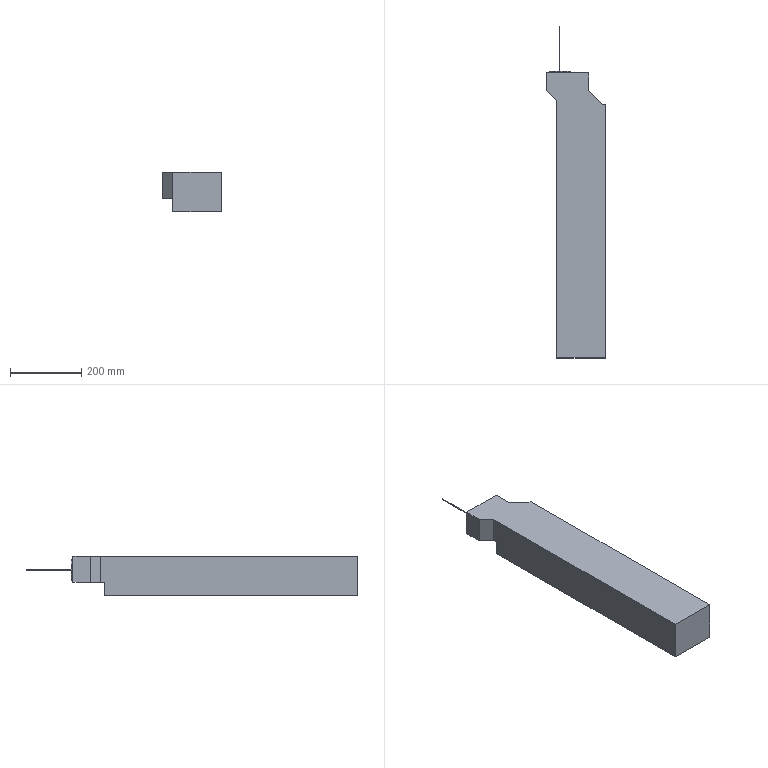Component | SolidWorks | 3120-HSC60-125-1 | 1 solid | 66 faces | volume 11654015 mm3 | cylinder 36 | plane 30 | commonest cylinder face diameters 6 x32 2 x2 60 x2